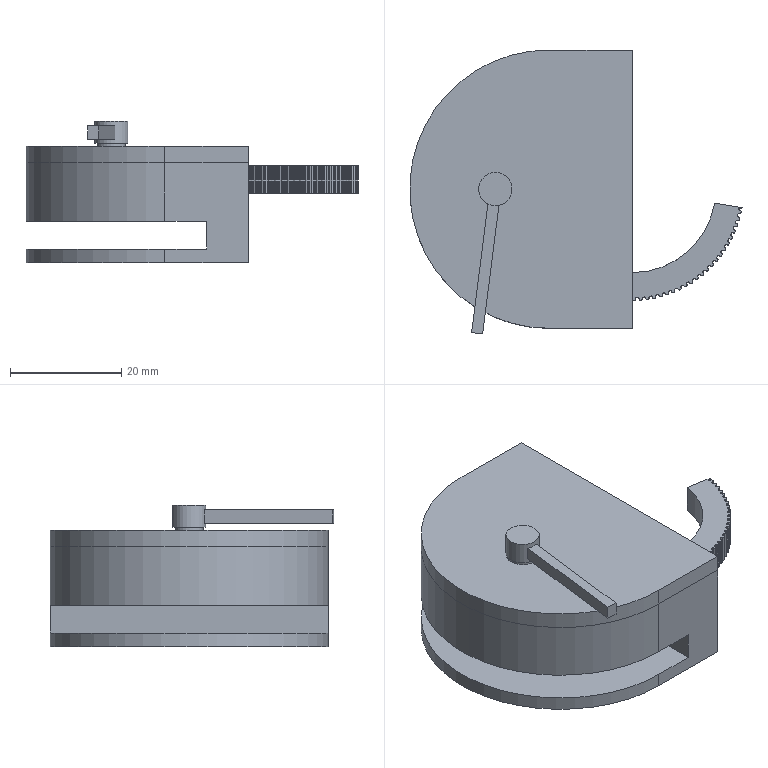Assembly | NX | mm | 5 component files | 5 solids | 705 faces | box 59.72 x 51.03 x 25.5 mm | volume 18142 mm3 | cylinder 478 | plane 227 | commonest cylinder face diameters 0.4 x300 40 x53 39 x52 10 x24 9 x24 30 x8 50 x3 28 x3
Bill of materials:
unnamed part 1 | 1 |  | Thin flat plate with a D-shaped outline (one semicircular edge, one straight edge) and a single small round through-hole near the center of the curved end.
unnamed part 2 | 1 |  | Straight arm with a rectangular cross-section, joined at one end to a short cylindrical hub. A small square/rectangular boss sticks out from the underside of the hub.
unnamed part 3 | 1 |  | Toothed disc with roughly 24 rounded teeth around its edge. A cylindrical hub stands up from one face, and the top of the hub has a square socket.
unnamed part 4 | 1 |  | Open, partial ring segment (about a C-shaped arc covering more than 180 degrees) with fine teeth around its outer edge and a smooth inner bore. One end has a stepped notch or hook on the inner side.
unnamed part 5 | 1 |  | Open-top housing with a D-shaped outline (semicircular wall plus a straight wall) and a stepped lip at the top rim. Inside are a small cylindrical post and curved internal ribs/walls. There is a long horizontal slot through the curved side wall and small rectangular openings with triangular features near the top of the straight wall.
Mates:
1. fix | housing 1 component
2. concentric | housing_cover 1 edge | housing 1 edge
3. concentric | internal_structure 1 edge | housing 1 edge
4. concentric | internal_gear 1 edge | housing 1 edge
5. touch align | handle 1 face | internal_gear 1 face
6. touch align | handle 1 face | internal_gear 1 face
7. touch align | handle 1 face | internal_gear 1 face